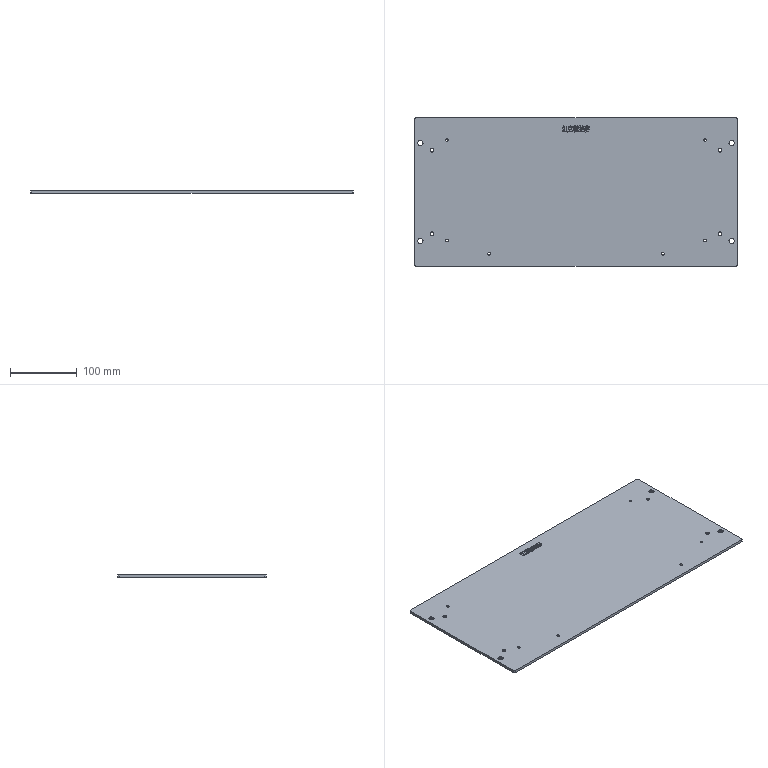CAM job | Mastercam | mm | 7 operations | part box 482.6 x 221.45 x 4
1. Contour (Ramp) | 9 - 10 平铣刀
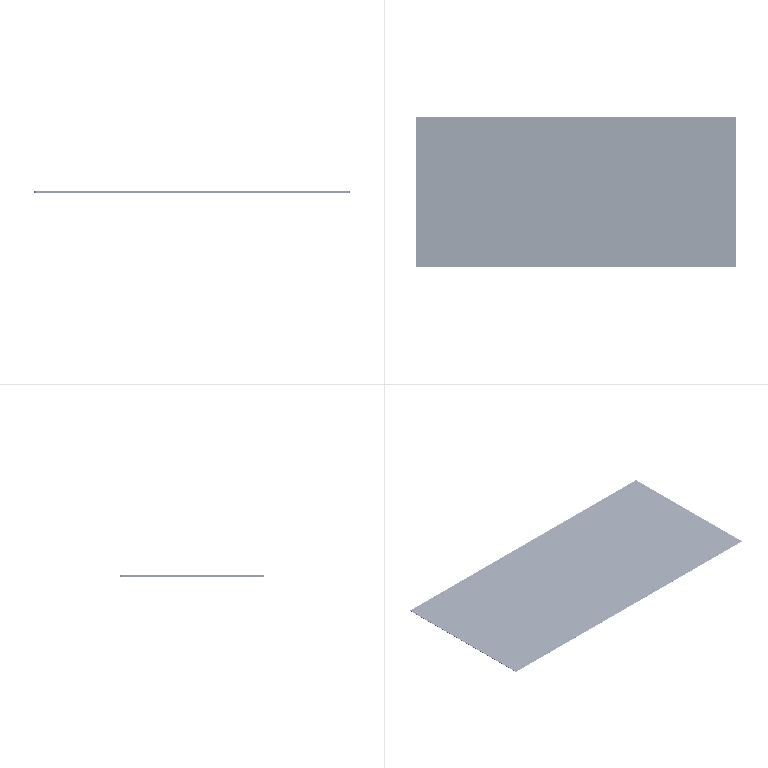2. Contour (2D) | 10 - 10 平铣刀
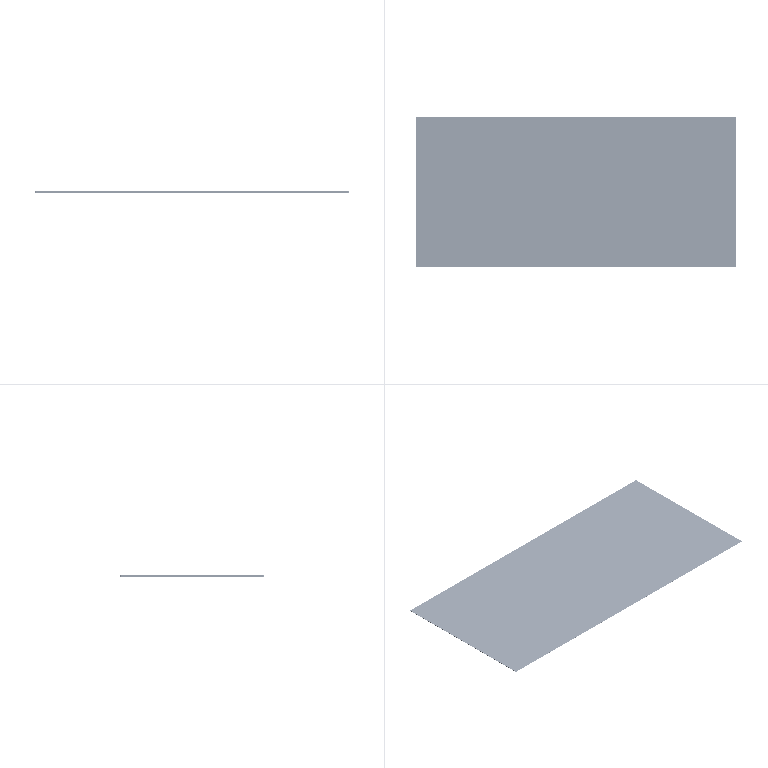3. Contour (Ramp) | 4 - 4 平铣刀
4. 3D High Speed (Waterline) | 14 - 4 圆鼻铣刀
5. Contour (2D) | 3 - 3 平铣刀
6. Drill/Counterbore | 7 - 4 倒角刀
7. Contour (2D chamfer) | 7 - 4 倒角刀